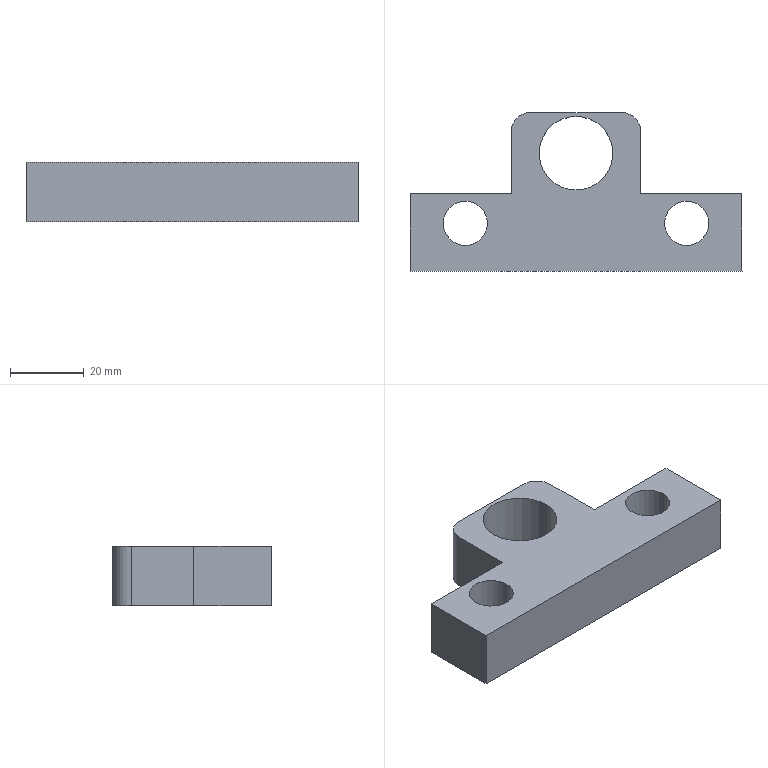Component | SolidWorks | NewTypeCurveBenderCylinderPlate-DoubleWheel-1 | 1 solid | 18 faces | box 90 x 43 x 16 mm | volume 33743 mm3 | plane 10 | cylinder 8 | commonest cylinder face diameters 12 x4 20 x2 10 x2
build123d program:
from build123d import *

# Parameters (mm, degrees)
SKETCH1_W           = 90
SKETCH1_H           = 43
BOSS_EXTRUDE1_DEPTH = 16
SKETCH2_R           = 10
SKETCH2_R_2         = 6
CUT_EXTRUDE1_DEPTH  = 53.376
SKETCH3_W           = 27.5
SKETCH3_H           = 22
CUT_EXTRUDE2_DEPTH  = 20
FILLET1_R           = 5


with BuildPart() as part:
    # Sketch1 → Boss-Extrude1 (new body)
    with BuildSketch(Plane.XY):
        Rectangle(SKETCH1_W, SKETCH1_H)
    extrude(amount=BOSS_EXTRUDE1_DEPTH)

    # Sketch2 → Cut-Extrude1 (cut, through all)
    with BuildSketch(Plane.XY.offset(16)):
        with Locations((0, -10.5)):
            Circle(SKETCH2_R)
        with Locations((-30, 8.5)):
            Circle(SKETCH2_R_2)
        with Locations(Location((30, 8.5, 0), (0, 0, 180))):
            Circle(SKETCH2_R_2)
    extrude(amount=-CUT_EXTRUDE1_DEPTH, mode=Mode.SUBTRACT)

    # Sketch3 → Cut-Extrude2 (cut)
    with BuildSketch(Plane.XY.offset(16)):
        with Locations((31.25, -10.5)):
            Rectangle(SKETCH3_W, SKETCH3_H)
        with Locations((-31.25, -10.5)):
            Rectangle(SKETCH3_W, SKETCH3_H)
    extrude(amount=-CUT_EXTRUDE2_DEPTH, mode=Mode.SUBTRACT)

    # Fillet1
    fillet1_edges = [part.edges().sort_by_distance(p)[0] for p in [
        (17.5, -21.5, 8),
        (-17.5, -21.5, 8),
    ]]
    fillet(fillet1_edges, radius=FILLET1_R)


solid = part.part

# Placed as in the assembly
solid = solid.moved(Location((0, 36.5, 226), (180, 0, 0)))
STEP:
#1=COLOUR_RGB('',0.7922,0.8196,0.9333);
#2=FILL_AREA_STYLE_COLOUR('',#1);
#3=FILL_AREA_STYLE('',(#2));
#4=SURFACE_STYLE_FILL_AREA(#3);
#5=SURFACE_SIDE_STYLE('',(#4));
#6=SURFACE_STYLE_USAGE(.BOTH.,#5);
#7=PRESENTATION_STYLE_ASSIGNMENT((#6));
#8=CARTESIAN_POINT('',(0.3937,1.85,8.268));
#9=VERTEX_POINT('',#8);
#10=CARTESIAN_POINT('',(-0.3937,1.85,8.268));
#11=VERTEX_POINT('',#10);
#12=CARTESIAN_POINT('',(-0.,1.85,8.268));
#13=DIRECTION('',(0.,-0.,1.));
#14=DIRECTION('',(-1.,0.,0.));
#15=AXIS2_PLACEMENT_3D('',#12,#13,#14);
#16=CIRCLE('',#15,0.3937);
#17=EDGE_CURVE('',#9,#11,#16,.T.);
#18=ORIENTED_EDGE('',*,*,#17,.F.);
#19=CARTESIAN_POINT('',(0.3937,1.85,8.898));
#20=VERTEX_POINT('',#19);
#21=CARTESIAN_POINT('',(0.3937,1.85,8.268));
#22=DIRECTION('',(0.,-0.,1.));
#23=VECTOR('',#22,39.37);
#24=LINE('',#21,#23);
#25=EDGE_CURVE('',#9,#20,#24,.T.);
#26=ORIENTED_EDGE('',*,*,#25,.T.);
#27=CARTESIAN_POINT('',(-0.3937,1.85,8.898));
#28=VERTEX_POINT('',#27);
#29=CARTESIAN_POINT('',(-0.,1.85,8.898));
#30=DIRECTION('',(0.,-0.,1.));
#31=DIRECTION('',(-1.,0.,0.));
#32=AXIS2_PLACEMENT_3D('',#29,#30,#31);
#33=CIRCLE('',#32,0.3937);
#34=EDGE_CURVE('',#20,#28,#33,.T.);
#35=ORIENTED_EDGE('',*,*,#34,.T.);
#36=CARTESIAN_POINT('',(-0.3937,1.85,8.268));
#37=DIRECTION('',(0.,-0.,1.));
#38=VECTOR('',#37,39.37);
#39=LINE('',#36,#38);
#40=EDGE_CURVE('',#11,#28,#39,.T.);
#41=ORIENTED_EDGE('',*,*,#40,.F.);
#42=EDGE_LOOP('',(#18,#26,#35,#41));
#43=FACE_OUTER_BOUND('',#42,.T.);
#44=CARTESIAN_POINT('',(-0.,1.85,8.268));
#45=DIRECTION('',(0.,-0.,1.));
#46=DIRECTION('',(-1.,0.,0.));
#47=AXIS2_PLACEMENT_3D('',#44,#45,#46);
#48=CYLINDRICAL_SURFACE('',#47,0.3937);
#49=ADVANCED_FACE('',(#43),#48,.F.);
#50=CARTESIAN_POINT('',(1.417,1.102,8.268));
#51=VERTEX_POINT('',#50);
#52=CARTESIAN_POINT('',(0.9449,1.102,8.268));
#53=VERTEX_POINT('',#52);
#54=CARTESIAN_POINT('',(1.181,1.102,8.268));
#55=DIRECTION('',(0.,-0.,1.));
#56=DIRECTION('',(-1.,0.,0.));
#57=AXIS2_PLACEMENT_3D('',#54,#55,#56);
#58=CIRCLE('',#57,0.2362);
#59=EDGE_CURVE('',#51,#53,#58,.T.);
#60=ORIENTED_EDGE('',*,*,#59,.F.);
#61=CARTESIAN_POINT('',(1.417,1.102,8.898));
#62=VERTEX_POINT('',#61);
#63=CARTESIAN_POINT('',(1.417,1.102,8.268));
#64=DIRECTION('',(0.,-0.,1.));
#65=VECTOR('',#64,39.37);
#66=LINE('',#63,#65);
#67=EDGE_CURVE('',#51,#62,#66,.T.);
#68=ORIENTED_EDGE('',*,*,#67,.T.);
#69=CARTESIAN_POINT('',(0.9449,1.102,8.898));
#70=VERTEX_POINT('',#69);
#71=CARTESIAN_POINT('',(1.181,1.102,8.898));
#72=DIRECTION('',(0.,-0.,1.));
#73=DIRECTION('',(-1.,0.,0.));
#74=AXIS2_PLACEMENT_3D('',#71,#72,#73);
#75=CIRCLE('',#74,0.2362);
#76=EDGE_CURVE('',#62,#70,#75,.T.);
#77=ORIENTED_EDGE('',*,*,#76,.T.);
#78=CARTESIAN_POINT('',(0.9449,1.102,8.268));
#79=DIRECTION('',(0.,-0.,1.));
#80=VECTOR('',#79,39.37);
#81=LINE('',#78,#80);
#82=EDGE_CURVE('',#53,#70,#81,.T.);
#83=ORIENTED_EDGE('',*,*,#82,.F.);
#84=EDGE_LOOP('',(#60,#68,#77,#83));
#85=FACE_OUTER_BOUND('',#84,.T.);
#86=CARTESIAN_POINT('',(1.181,1.102,8.268));
#87=DIRECTION('',(0.,-0.,1.));
#88=DIRECTION('',(-1.,0.,0.));
#89=AXIS2_PLACEMENT_3D('',#86,#87,#88);
#90=CYLINDRICAL_SURFACE('',#89,0.2362);
#91=ADVANCED_FACE('',(#85),#90,.F.);
#92=CARTESIAN_POINT('',(-0.9449,1.102,8.268));
#93=VERTEX_POINT('',#92);
#94=CARTESIAN_POINT('',(-1.417,1.102,8.268));
#95=VERTEX_POINT('',#94);
#96=CARTESIAN_POINT('',(-1.181,1.102,8.268));
#97=DIRECTION('',(0.,-0.,1.));
#98=DIRECTION('',(1.,0.,0.));
#99=AXIS2_PLACEMENT_3D('',#96,#97,#98);
#100=CIRCLE('',#99,0.2362);
#101=EDGE_CURVE('',#93,#95,#100,.T.);
#102=ORIENTED_EDGE('',*,*,#101,.F.);
#103=CARTESIAN_POINT('',(-0.9449,1.102,8.898));
#104=VERTEX_POINT('',#103);
#105=CARTESIAN_POINT('',(-0.9449,1.102,8.268));
#106=DIRECTION('',(0.,-0.,1.));
#107=VECTOR('',#106,39.37);
#108=LINE('',#105,#107);
#109=EDGE_CURVE('',#93,#104,#108,.T.);
#110=ORIENTED_EDGE('',*,*,#109,.T.);
#111=CARTESIAN_POINT('',(-1.417,1.102,8.898));
#112=VERTEX_POINT('',#111);
#113=CARTESIAN_POINT('',(-1.181,1.102,8.898));
#114=DIRECTION('',(0.,-0.,1.));
#115=DIRECTION('',(1.,0.,0.));
#116=AXIS2_PLACEMENT_3D('',#113,#114,#115);
#117=CIRCLE('',#116,0.2362);
#118=EDGE_CURVE('',#104,#112,#117,.T.);
#119=ORIENTED_EDGE('',*,*,#118,.T.);
#120=CARTESIAN_POINT('',(-1.417,1.102,8.268));
#121=DIRECTION('',(0.,-0.,1.));
#122=VECTOR('',#121,39.37);
#123=LINE('',#120,#122);
#124=EDGE_CURVE('',#95,#112,#123,.T.);
#125=ORIENTED_EDGE('',*,*,#124,.F.);
#126=EDGE_LOOP('',(#102,#110,#119,#125));
#127=FACE_OUTER_BOUND('',#126,.T.);
#128=CARTESIAN_POINT('',(-1.181,1.102,8.268));
#129=DIRECTION('',(0.,-0.,1.));
#130=DIRECTION('',(-1.,0.,0.));
#131=AXIS2_PLACEMENT_3D('',#128,#129,#130);
#132=CYLINDRICAL_SURFACE('',#131,0.2362);
#133=ADVANCED_FACE('',(#127),#132,.F.);
#134=CARTESIAN_POINT('',(-1.772,1.417,8.898));
#135=VERTEX_POINT('',#134);
#136=CARTESIAN_POINT('',(-1.772,0.5906,8.898));
#137=VERTEX_POINT('',#136);
#138=CARTESIAN_POINT('',(-1.772,0.5906,8.898));
#139=DIRECTION('',(0.,-1.,-0.));
#140=VECTOR('',#139,39.37);
#141=LINE('',#138,#140);
#142=EDGE_CURVE('',#135,#137,#141,.T.);
#143=ORIENTED_EDGE('',*,*,#142,.F.);
#144=CARTESIAN_POINT('',(-1.772,1.417,8.268));
#145=VERTEX_POINT('',#144);
#146=CARTESIAN_POINT('',(-1.772,1.417,8.11));
#147=DIRECTION('',(0.,-0.,1.));
#148=VECTOR('',#147,39.37);
#149=LINE('',#146,#148);
#150=EDGE_CURVE('',#145,#135,#149,.T.);
#151=ORIENTED_EDGE('',*,*,#150,.F.);
#152=CARTESIAN_POINT('',(-1.772,0.5906,8.268));
#153=VERTEX_POINT('',#152);
#154=CARTESIAN_POINT('',(-1.772,0.5906,8.268));
#155=DIRECTION('',(0.,-1.,-0.));
#156=VECTOR('',#155,39.37);
#157=LINE('',#154,#156);
#158=EDGE_CURVE('',#145,#153,#157,.T.);
#159=ORIENTED_EDGE('',*,*,#158,.T.);
#160=CARTESIAN_POINT('',(-1.772,0.5906,8.898));
#161=DIRECTION('',(-0.,0.,-1.));
#162=VECTOR('',#161,39.37);
#163=LINE('',#160,#162);
#164=EDGE_CURVE('',#137,#153,#163,.T.);
#165=ORIENTED_EDGE('',*,*,#164,.F.);
#166=EDGE_LOOP('',(#143,#151,#159,#165));
#167=FACE_OUTER_BOUND('',#166,.T.);
#168=CARTESIAN_POINT('',(-1.772,0.5906,8.898));
#169=DIRECTION('',(1.,0.,-0.));
#170=DIRECTION('',(-0.,1.,0.));
#171=AXIS2_PLACEMENT_3D('',#168,#169,#170);
#172=PLANE('',#171);
#173=ADVANCED_FACE('',(#167),#172,.F.);
#174=CARTESIAN_POINT('',(1.772,0.5906,8.268));
#175=VERTEX_POINT('',#174);
#176=CARTESIAN_POINT('',(1.772,0.5906,8.268));
#177=DIRECTION('',(1.,-0.,-0.));
#178=VECTOR('',#177,39.37);
#179=LINE('',#176,#178);
#180=EDGE_CURVE('',#153,#175,#179,.T.);
#181=ORIENTED_EDGE('',*,*,#180,.T.);
#182=CARTESIAN_POINT('',(1.772,0.5906,8.898));
#183=VERTEX_POINT('',#182);
#184=CARTESIAN_POINT('',(1.772,0.5906,8.898));
#185=DIRECTION('',(-0.,0.,-1.));
#186=VECTOR('',#185,39.37);
#187=LINE('',#184,#186);
#188=EDGE_CURVE('',#183,#175,#187,.T.);
#189=ORIENTED_EDGE('',*,*,#188,.F.);
#190=CARTESIAN_POINT('',(1.772,0.5906,8.898));
#191=DIRECTION('',(1.,-0.,-0.));
#192=VECTOR('',#191,39.37);
#193=LINE('',#190,#192);
#194=EDGE_CURVE('',#137,#183,#193,.T.);
#195=ORIENTED_EDGE('',*,*,#194,.F.);
#196=ORIENTED_EDGE('',*,*,#164,.T.);
#197=EDGE_LOOP('',(#181,#189,#195,#196));
#198=FACE_OUTER_BOUND('',#197,.T.);
#199=CARTESIAN_POINT('',(1.772,0.5906,8.898));
#200=DIRECTION('',(-0.,1.,0.));
#201=DIRECTION('',(-0.,0.,-1.));
#202=AXIS2_PLACEMENT_3D('',#199,#200,#201);
#203=PLANE('',#202);
#204=ADVANCED_FACE('',(#198),#203,.F.);
#205=CARTESIAN_POINT('',(1.772,1.417,8.268));
#206=VERTEX_POINT('',#205);
#207=CARTESIAN_POINT('',(1.772,0.5906,8.268));
#208=DIRECTION('',(-0.,1.,0.));
#209=VECTOR('',#208,39.37);
#210=LINE('',#207,#209);
#211=EDGE_CURVE('',#175,#206,#210,.T.);
#212=ORIENTED_EDGE('',*,*,#211,.T.);
#213=CARTESIAN_POINT('',(1.772,1.417,8.898));
#214=VERTEX_POINT('',#213);
#215=CARTESIAN_POINT('',(1.772,1.417,8.11));
#216=DIRECTION('',(0.,-0.,1.));
#217=VECTOR('',#216,39.37);
#218=LINE('',#215,#217);
#219=EDGE_CURVE('',#206,#214,#218,.T.);
#220=ORIENTED_EDGE('',*,*,#219,.T.);
#221=CARTESIAN_POINT('',(1.772,0.5906,8.898));
#222=DIRECTION('',(-0.,1.,0.));
#223=VECTOR('',#222,39.37);
#224=LINE('',#221,#223);
#225=EDGE_CURVE('',#183,#214,#224,.T.);
#226=ORIENTED_EDGE('',*,*,#225,.F.);
#227=ORIENTED_EDGE('',*,*,#188,.T.);
#228=EDGE_LOOP('',(#212,#220,#226,#227));
#229=FACE_OUTER_BOUND('',#228,.T.);
#230=CARTESIAN_POINT('',(1.772,0.5906,8.898));
#231=DIRECTION('',(-1.,-0.,0.));
#232=DIRECTION('',(0.,-1.,-0.));
#233=AXIS2_PLACEMENT_3D('',#230,#231,#232);
#234=PLANE('',#233);
#235=ADVANCED_FACE('',(#229),#234,.F.);
#236=CARTESIAN_POINT('',(0.4921,2.283,8.268));
#237=VERTEX_POINT('',#236);
#238=CARTESIAN_POINT('',(-0.4921,2.283,8.268));
#239=VERTEX_POINT('',#238);
#240=CARTESIAN_POINT('',(1.772,2.283,8.268));
#241=DIRECTION('',(-1.,0.,0.));
#242=VECTOR('',#241,39.37);
#243=LINE('',#240,#242);
#244=EDGE_CURVE('',#237,#239,#243,.T.);
#245=ORIENTED_EDGE('',*,*,#244,.T.);
#246=CARTESIAN_POINT('',(-0.4921,2.283,8.898));
#247=VERTEX_POINT('',#246);
#248=CARTESIAN_POINT('',(-0.4921,2.283,8.898));
#249=DIRECTION('',(0.,-0.,1.));
#250=VECTOR('',#249,39.37);
#251=LINE('',#248,#250);
#252=EDGE_CURVE('',#239,#247,#251,.T.);
#253=ORIENTED_EDGE('',*,*,#252,.T.);
#254=CARTESIAN_POINT('',(0.4921,2.283,8.898));
#255=VERTEX_POINT('',#254);
#256=CARTESIAN_POINT('',(1.772,2.283,8.898));
#257=DIRECTION('',(-1.,0.,0.));
#258=VECTOR('',#257,39.37);
#259=LINE('',#256,#258);
#260=EDGE_CURVE('',#255,#247,#259,.T.);
#261=ORIENTED_EDGE('',*,*,#260,.F.);
#262=CARTESIAN_POINT('',(0.4921,2.283,8.898));
#263=DIRECTION('',(-0.,0.,-1.));
#264=VECTOR('',#263,39.37);
#265=LINE('',#262,#264);
#266=EDGE_CURVE('',#255,#237,#265,.T.);
#267=ORIENTED_EDGE('',*,*,#266,.T.);
#268=EDGE_LOOP('',(#245,#253,#261,#267));
#269=FACE_OUTER_BOUND('',#268,.T.);
#270=CARTESIAN_POINT('',(1.772,2.283,8.898));
#271=DIRECTION('',(0.,-1.,-0.));
#272=DIRECTION('',(0.,-0.,1.));
#273=AXIS2_PLACEMENT_3D('',#270,#271,#272);
#274=PLANE('',#273);
#275=ADVANCED_FACE('',(#269),#274,.F.);
#276=ORIENTED_EDGE('',*,*,#260,.T.);
#277=CARTESIAN_POINT('',(-0.689,2.087,8.898));
#278=VERTEX_POINT('',#277);
#279=CARTESIAN_POINT('',(-0.4921,2.087,8.898));
#280=DIRECTION('',(0.,-0.,1.));
#281=DIRECTION('',(-1.,0.,0.));
#282=AXIS2_PLACEMENT_3D('',#279,#280,#281);
#283=CIRCLE('',#282,0.1969);
#284=EDGE_CURVE('',#247,#278,#283,.T.);
#285=ORIENTED_EDGE('',*,*,#284,.T.);
#286=CARTESIAN_POINT('',(-0.689,1.417,8.898));
#287=VERTEX_POINT('',#286);
#288=CARTESIAN_POINT('',(-0.689,1.417,8.898));
#289=DIRECTION('',(-0.,1.,0.));
#290=VECTOR('',#289,39.37);
#291=LINE('',#288,#290);
#292=EDGE_CURVE('',#287,#278,#291,.T.);
#293=ORIENTED_EDGE('',*,*,#292,.F.);
#294=CARTESIAN_POINT('',(-1.772,1.417,8.898));
#295=DIRECTION('',(1.,-0.,-0.));
#296=VECTOR('',#295,39.37);
#297=LINE('',#294,#296);
#298=EDGE_CURVE('',#135,#287,#297,.T.);
#299=ORIENTED_EDGE('',*,*,#298,.F.);
#300=ORIENTED_EDGE('',*,*,#142,.T.);
#301=ORIENTED_EDGE('',*,*,#194,.T.);
#302=ORIENTED_EDGE('',*,*,#225,.T.);
#303=CARTESIAN_POINT('',(0.689,1.417,8.898));
#304=VERTEX_POINT('',#303);
#305=CARTESIAN_POINT('',(1.772,1.417,8.898));
#306=DIRECTION('',(1.,0.,-0.));
#307=VECTOR('',#306,39.37);
#308=LINE('',#305,#307);
#309=EDGE_CURVE('',#304,#214,#308,.T.);
#310=ORIENTED_EDGE('',*,*,#309,.F.);
#311=CARTESIAN_POINT('',(0.689,2.087,8.898));
#312=VERTEX_POINT('',#311);
#313=CARTESIAN_POINT('',(0.689,1.417,8.898));
#314=DIRECTION('',(0.,-1.,-0.));
#315=VECTOR('',#314,39.37);
#316=LINE('',#313,#315);
#317=EDGE_CURVE('',#312,#304,#316,.T.);
#318=ORIENTED_EDGE('',*,*,#317,.F.);
#319=CARTESIAN_POINT('',(0.4921,2.087,8.898));
#320=DIRECTION('',(0.,-0.,1.));
#321=DIRECTION('',(-1.,0.,0.));
#322=AXIS2_PLACEMENT_3D('',#319,#320,#321);
#323=CIRCLE('',#322,0.1969);
#324=EDGE_CURVE('',#312,#255,#323,.T.);
#325=ORIENTED_EDGE('',*,*,#324,.T.);
#326=EDGE_LOOP('',(#276,#285,#293,#299,#300,#301,#302,#310,#318,#325));
#327=FACE_OUTER_BOUND('',#326,.T.);
#328=CARTESIAN_POINT('',(-0.,1.85,8.898));
#329=DIRECTION('',(0.,-0.,1.));
#330=DIRECTION('',(-1.,0.,0.));
#331=AXIS2_PLACEMENT_3D('',#328,#329,#330);
#332=CIRCLE('',#331,0.3937);
#333=EDGE_CURVE('',#28,#20,#332,.T.);
#334=ORIENTED_EDGE('',*,*,#333,.F.);
#335=ORIENTED_EDGE('',*,*,#34,.F.);
#336=EDGE_LOOP('',(#334,#335));
#337=FACE_BOUND('',#336,.T.);
#338=CARTESIAN_POINT('',(1.181,1.102,8.898));
#339=DIRECTION('',(0.,-0.,1.));
#340=DIRECTION('',(-1.,0.,0.));
#341=AXIS2_PLACEMENT_3D('',#338,#339,#340);
#342=CIRCLE('',#341,0.2362);
#343=EDGE_CURVE('',#70,#62,#342,.T.);
#344=ORIENTED_EDGE('',*,*,#343,.F.);
#345=ORIENTED_EDGE('',*,*,#76,.F.);
#346=EDGE_LOOP('',(#344,#345));
#347=FACE_BOUND('',#346,.T.);
#348=CARTESIAN_POINT('',(-1.181,1.102,8.898));
#349=DIRECTION('',(0.,-0.,1.));
#350=DIRECTION('',(1.,0.,0.));
#351=AXIS2_PLACEMENT_3D('',#348,#349,#350);
#352=CIRCLE('',#351,0.2362);
#353=EDGE_CURVE('',#112,#104,#352,.T.);
#354=ORIENTED_EDGE('',*,*,#353,.F.);
#355=ORIENTED_EDGE('',*,*,#118,.F.);
#356=EDGE_LOOP('',(#354,#355));
#357=FACE_BOUND('',#356,.T.);
#358=CARTESIAN_POINT('',(-0.,1.437,8.898));
#359=DIRECTION('',(0.,-0.,1.));
#360=DIRECTION('',(-1.,0.,0.));
#361=AXIS2_PLACEMENT_3D('',#358,#359,#360);
#362=PLANE('',#361);
#363=ADVANCED_FACE('',(#327,#337,#347,#357),#362,.T.);
#364=CARTESIAN_POINT('',(-0.,1.85,8.268));
#365=DIRECTION('',(0.,-0.,1.));
#366=DIRECTION('',(-1.,0.,0.));
#367=AXIS2_PLACEMENT_3D('',#364,#365,#366);
#368=CIRCLE('',#367,0.3937);
#369=EDGE_CURVE('',#11,#9,#368,.T.);
#370=ORIENTED_EDGE('',*,*,#369,.T.);
#371=ORIENTED_EDGE('',*,*,#17,.T.);
#372=EDGE_LOOP('',(#370,#371));
#373=FACE_BOUND('',#372,.T.);
#374=CARTESIAN_POINT('',(1.181,1.102,8.268));
#375=DIRECTION('',(0.,-0.,1.));
#376=DIRECTION('',(-1.,0.,0.));
#377=AXIS2_PLACEMENT_3D('',#374,#375,#376);
#378=CIRCLE('',#377,0.2362);
#379=EDGE_CURVE('',#53,#51,#378,.T.);
#380=ORIENTED_EDGE('',*,*,#379,.T.);
#381=ORIENTED_EDGE('',*,*,#59,.T.);
#382=EDGE_LOOP('',(#380,#381));
#383=FACE_BOUND('',#382,.T.);
#384=CARTESIAN_POINT('',(-1.181,1.102,8.268));
#385=DIRECTION('',(0.,-0.,1.));
#386=DIRECTION('',(1.,0.,0.));
#387=AXIS2_PLACEMENT_3D('',#384,#385,#386);
#388=CIRCLE('',#387,0.2362);
#389=EDGE_CURVE('',#95,#93,#388,.T.);
#390=ORIENTED_EDGE('',*,*,#389,.T.);
#391=ORIENTED_EDGE('',*,*,#101,.T.);
#392=EDGE_LOOP('',(#390,#391));
#393=FACE_BOUND('',#392,.T.);
#394=CARTESIAN_POINT('',(-0.689,1.417,8.268));
#395=VERTEX_POINT('',#394);
#396=CARTESIAN_POINT('',(-0.689,2.087,8.268));
#397=VERTEX_POINT('',#396);
#398=CARTESIAN_POINT('',(-0.689,1.437,8.268));
#399=DIRECTION('',(-0.,1.,0.));
#400=VECTOR('',#399,39.37);
#401=LINE('',#398,#400);
#402=EDGE_CURVE('',#395,#397,#401,.T.);
#403=ORIENTED_EDGE('',*,*,#402,.T.);
#404=CARTESIAN_POINT('',(-0.4921,2.087,8.268));
#405=DIRECTION('',(-0.,0.,-1.));
#406=DIRECTION('',(-1.,0.,0.));
#407=AXIS2_PLACEMENT_3D('',#404,#405,#406);
#408=CIRCLE('',#407,0.1969);
#409=EDGE_CURVE('',#397,#239,#408,.T.);
#410=ORIENTED_EDGE('',*,*,#409,.T.);
#411=ORIENTED_EDGE('',*,*,#244,.F.);
#412=CARTESIAN_POINT('',(0.689,2.087,8.268));
#413=VERTEX_POINT('',#412);
#414=CARTESIAN_POINT('',(0.4921,2.087,8.268));
#415=DIRECTION('',(-0.,0.,-1.));
#416=DIRECTION('',(-1.,-0.,0.));
#417=AXIS2_PLACEMENT_3D('',#414,#415,#416);
#418=CIRCLE('',#417,0.1969);
#419=EDGE_CURVE('',#237,#413,#418,.T.);
#420=ORIENTED_EDGE('',*,*,#419,.T.);
#421=CARTESIAN_POINT('',(0.689,1.417,8.268));
#422=VERTEX_POINT('',#421);
#423=CARTESIAN_POINT('',(0.689,1.437,8.268));
#424=DIRECTION('',(0.,-1.,-0.));
#425=VECTOR('',#424,39.37);
#426=LINE('',#423,#425);
#427=EDGE_CURVE('',#413,#422,#426,.T.);
#428=ORIENTED_EDGE('',*,*,#427,.T.);
#429=CARTESIAN_POINT('',(-0.,1.417,8.268));
#430=DIRECTION('',(1.,0.,-0.));
#431=VECTOR('',#430,39.37);
#432=LINE('',#429,#431);
#433=EDGE_CURVE('',#422,#206,#432,.T.);
#434=ORIENTED_EDGE('',*,*,#433,.T.);
#435=ORIENTED_EDGE('',*,*,#211,.F.);
#436=ORIENTED_EDGE('',*,*,#180,.F.);
#437=ORIENTED_EDGE('',*,*,#158,.F.);
#438=CARTESIAN_POINT('',(-0.,1.417,8.268));
#439=DIRECTION('',(1.,-0.,-0.));
#440=VECTOR('',#439,39.37);
#441=LINE('',#438,#440);
#442=EDGE_CURVE('',#145,#395,#441,.T.);
#443=ORIENTED_EDGE('',*,*,#442,.T.);
#444=EDGE_LOOP('',(#403,#410,#411,#420,#428,#434,#435,#436,#437,#443));
#445=FACE_OUTER_BOUND('',#444,.T.);
#446=CARTESIAN_POINT('',(-0.,1.437,8.268));
#447=DIRECTION('',(0.,-0.,1.));
#448=DIRECTION('',(-1.,0.,0.));
#449=AXIS2_PLACEMENT_3D('',#446,#447,#448);
#450=PLANE('',#449);
#451=ADVANCED_FACE('',(#373,#383,#393,#445),#450,.F.);
#452=ORIENTED_EDGE('',*,*,#109,.F.);
#453=ORIENTED_EDGE('',*,*,#389,.F.);
#454=ORIENTED_EDGE('',*,*,#124,.T.);
#455=ORIENTED_EDGE('',*,*,#353,.T.);
#456=EDGE_LOOP('',(#452,#453,#454,#455));
#457=FACE_OUTER_BOUND('',#456,.T.);
#458=CARTESIAN_POINT('',(-1.181,1.102,8.268));
#459=DIRECTION('',(0.,-0.,1.));
#460=DIRECTION('',(-1.,0.,0.));
#461=AXIS2_PLACEMENT_3D('',#458,#459,#460);
#462=CYLINDRICAL_SURFACE('',#461,0.2362);
#463=ADVANCED_FACE('',(#457),#462,.F.);
#464=ORIENTED_EDGE('',*,*,#67,.F.);
#465=ORIENTED_EDGE('',*,*,#379,.F.);
#466=ORIENTED_EDGE('',*,*,#82,.T.);
#467=ORIENTED_EDGE('',*,*,#343,.T.);
#468=EDGE_LOOP('',(#464,#465,#466,#467));
#469=FACE_OUTER_BOUND('',#468,.T.);
#470=CARTESIAN_POINT('',(1.181,1.102,8.268));
#471=DIRECTION('',(0.,-0.,1.));
#472=DIRECTION('',(-1.,0.,0.));
#473=AXIS2_PLACEMENT_3D('',#470,#471,#472);
#474=CYLINDRICAL_SURFACE('',#473,0.2362);
#475=ADVANCED_FACE('',(#469),#474,.F.);
#476=ORIENTED_EDGE('',*,*,#25,.F.);
#477=ORIENTED_EDGE('',*,*,#369,.F.);
#478=ORIENTED_EDGE('',*,*,#40,.T.);
#479=ORIENTED_EDGE('',*,*,#333,.T.);
#480=EDGE_LOOP('',(#476,#477,#478,#479));
#481=FACE_OUTER_BOUND('',#480,.T.);
#482=CARTESIAN_POINT('',(-0.,1.85,8.268));
#483=DIRECTION('',(0.,-0.,1.));
#484=DIRECTION('',(-1.,0.,0.));
#485=AXIS2_PLACEMENT_3D('',#482,#483,#484);
#486=CYLINDRICAL_SURFACE('',#485,0.3937);
#487=ADVANCED_FACE('',(#481),#486,.F.);
#488=CARTESIAN_POINT('',(0.689,1.417,8.11));
#489=DIRECTION('',(0.,-0.,1.));
#490=VECTOR('',#489,39.37);
#491=LINE('',#488,#490);
#492=EDGE_CURVE('',#422,#304,#491,.T.);
#493=ORIENTED_EDGE('',*,*,#492,.T.);
#494=ORIENTED_EDGE('',*,*,#309,.T.);
#495=ORIENTED_EDGE('',*,*,#219,.F.);
#496=ORIENTED_EDGE('',*,*,#433,.F.);
#497=EDGE_LOOP('',(#493,#494,#495,#496));
#498=FACE_OUTER_BOUND('',#497,.T.);
#499=CARTESIAN_POINT('',(1.772,1.417,8.11));
#500=DIRECTION('',(0.,-1.,-0.));
#501=DIRECTION('',(1.,0.,-0.));
#502=AXIS2_PLACEMENT_3D('',#499,#500,#501);
#503=PLANE('',#502);
#504=ADVANCED_FACE('',(#498),#503,.F.);
#505=ORIENTED_EDGE('',*,*,#427,.F.);
#506=CARTESIAN_POINT('',(0.689,2.087,8.11));
#507=DIRECTION('',(0.,-0.,1.));
#508=VECTOR('',#507,39.37);
#509=LINE('',#506,#508);
#510=EDGE_CURVE('',#413,#312,#509,.T.);
#511=ORIENTED_EDGE('',*,*,#510,.T.);
#512=ORIENTED_EDGE('',*,*,#317,.T.);
#513=ORIENTED_EDGE('',*,*,#492,.F.);
#514=EDGE_LOOP('',(#505,#511,#512,#513));
#515=FACE_OUTER_BOUND('',#514,.T.);
#516=CARTESIAN_POINT('',(0.689,1.417,8.11));
#517=DIRECTION('',(-1.,-0.,0.));
#518=DIRECTION('',(0.,-1.,-0.));
#519=AXIS2_PLACEMENT_3D('',#516,#517,#518);
#520=PLANE('',#519);
#521=ADVANCED_FACE('',(#515),#520,.F.);
#522=ORIENTED_EDGE('',*,*,#292,.T.);
#523=CARTESIAN_POINT('',(-0.689,2.087,8.11));
#524=DIRECTION('',(-0.,0.,-1.));
#525=VECTOR('',#524,39.37);
#526=LINE('',#523,#525);
#527=EDGE_CURVE('',#278,#397,#526,.T.);
#528=ORIENTED_EDGE('',*,*,#527,.T.);
#529=ORIENTED_EDGE('',*,*,#402,.F.);
#530=CARTESIAN_POINT('',(-0.689,1.417,8.11));
#531=DIRECTION('',(0.,-0.,1.));
#532=VECTOR('',#531,39.37);
#533=LINE('',#530,#532);
#534=EDGE_CURVE('',#395,#287,#533,.T.);
#535=ORIENTED_EDGE('',*,*,#534,.T.);
#536=EDGE_LOOP('',(#522,#528,#529,#535));
#537=FACE_OUTER_BOUND('',#536,.T.);
#538=CARTESIAN_POINT('',(-0.689,1.417,8.11));
#539=DIRECTION('',(1.,0.,-0.));
#540=DIRECTION('',(-0.,1.,0.));
#541=AXIS2_PLACEMENT_3D('',#538,#539,#540);
#542=PLANE('',#541);
#543=ADVANCED_FACE('',(#537),#542,.F.);
#544=ORIENTED_EDGE('',*,*,#150,.T.);
#545=ORIENTED_EDGE('',*,*,#298,.T.);
#546=ORIENTED_EDGE('',*,*,#534,.F.);
#547=ORIENTED_EDGE('',*,*,#442,.F.);
#548=EDGE_LOOP('',(#544,#545,#546,#547));
#549=FACE_OUTER_BOUND('',#548,.T.);
#550=CARTESIAN_POINT('',(-1.772,1.417,8.11));
#551=DIRECTION('',(-0.,-1.,-0.));
#552=DIRECTION('',(1.,-0.,-0.));
#553=AXIS2_PLACEMENT_3D('',#550,#551,#552);
#554=PLANE('',#553);
#555=ADVANCED_FACE('',(#549),#554,.F.);
#556=ORIENTED_EDGE('',*,*,#409,.F.);
#557=ORIENTED_EDGE('',*,*,#527,.F.);
#558=ORIENTED_EDGE('',*,*,#284,.F.);
#559=ORIENTED_EDGE('',*,*,#252,.F.);
#560=EDGE_LOOP('',(#556,#557,#558,#559));
#561=FACE_OUTER_BOUND('',#560,.T.);
#562=CARTESIAN_POINT('',(-0.4921,2.087,8.898));
#563=DIRECTION('',(0.,-0.,1.));
#564=DIRECTION('',(-1.,0.,0.));
#565=AXIS2_PLACEMENT_3D('',#562,#563,#564);
#566=CYLINDRICAL_SURFACE('',#565,0.1969);
#567=ADVANCED_FACE('',(#561),#566,.T.);
#568=ORIENTED_EDGE('',*,*,#419,.F.);
#569=ORIENTED_EDGE('',*,*,#266,.F.);
#570=ORIENTED_EDGE('',*,*,#324,.F.);
#571=ORIENTED_EDGE('',*,*,#510,.F.);
#572=EDGE_LOOP('',(#568,#569,#570,#571));
#573=FACE_OUTER_BOUND('',#572,.T.);
#574=CARTESIAN_POINT('',(0.4921,2.087,8.11));
#575=DIRECTION('',(0.,-0.,1.));
#576=DIRECTION('',(-1.,0.,0.));
#577=AXIS2_PLACEMENT_3D('',#574,#575,#576);
#578=CYLINDRICAL_SURFACE('',#577,0.1969);
#579=ADVANCED_FACE('',(#573),#578,.T.);
#580=CLOSED_SHELL('',(#49,#91,#133,#173,#204,#235,#275,#363,#451,#463,#475,#487,#504,#521,#543,#555,#567,#579));
#581=MANIFOLD_SOLID_BREP('',#580);
#582=STYLED_ITEM('',(#7),#581);
#583=PRESENTATION_LAYER_ASSIGNMENT('','',(#582));
#584=(LENGTH_UNIT()NAMED_UNIT(*)SI_UNIT($,.METRE.));
#585=LENGTH_MEASURE_WITH_UNIT(LENGTH_MEASURE(0.0254),#584);
#586=DIMENSIONAL_EXPONENTS(1.,0.,0.,0.,0.,0.,0.);
#587=(CONVERSION_BASED_UNIT('',#585)LENGTH_UNIT()NAMED_UNIT(#586));
#588=UNCERTAINTY_MEASURE_WITH_UNIT(LENGTH_MEASURE(0.00001),#587,'','');
#589=(NAMED_UNIT(*)PLANE_ANGLE_UNIT()SI_UNIT($,.RADIAN.));
#590=(NAMED_UNIT(*)SI_UNIT($,.STERADIAN.)SOLID_ANGLE_UNIT());
#591=(GEOMETRIC_REPRESENTATION_CONTEXT(3)GLOBAL_UNCERTAINTY_ASSIGNED_CONTEXT((#588))GLOBAL_UNIT_ASSIGNED_CONTEXT((#587,#589,#590))REPRESENTATION_CONTEXT('',''));
#592=MECHANICAL_DESIGN_GEOMETRIC_PRESENTATION_REPRESENTATION('',(#582),#591);
#593=CARTESIAN_POINT('',(0.,0.,0.));
#594=DIRECTION('',(0.,0.,1.));
#595=DIRECTION('',(1.,0.,0.));
#596=AXIS2_PLACEMENT_3D('',#593,#594,#595);
#597=(LENGTH_UNIT()NAMED_UNIT(*)SI_UNIT($,.METRE.));
#598=LENGTH_MEASURE_WITH_UNIT(LENGTH_MEASURE(0.0254),#597);
#599=DIMENSIONAL_EXPONENTS(1.,0.,0.,0.,0.,0.,0.);
#600=(CONVERSION_BASED_UNIT('',#598)LENGTH_UNIT()NAMED_UNIT(#599));
#601=UNCERTAINTY_MEASURE_WITH_UNIT(LENGTH_MEASURE(0.00001),#600,'','');
#602=(NAMED_UNIT(*)PLANE_ANGLE_UNIT()SI_UNIT($,.RADIAN.));
#603=(NAMED_UNIT(*)SI_UNIT($,.STERADIAN.)SOLID_ANGLE_UNIT());
#604=(GEOMETRIC_REPRESENTATION_CONTEXT(3)GLOBAL_UNCERTAINTY_ASSIGNED_CONTEXT((#601))GLOBAL_UNIT_ASSIGNED_CONTEXT((#600,#602,#603))REPRESENTATION_CONTEXT('',''));
#605=ADVANCED_BREP_SHAPE_REPRESENTATION('',(#581,#596),#604);